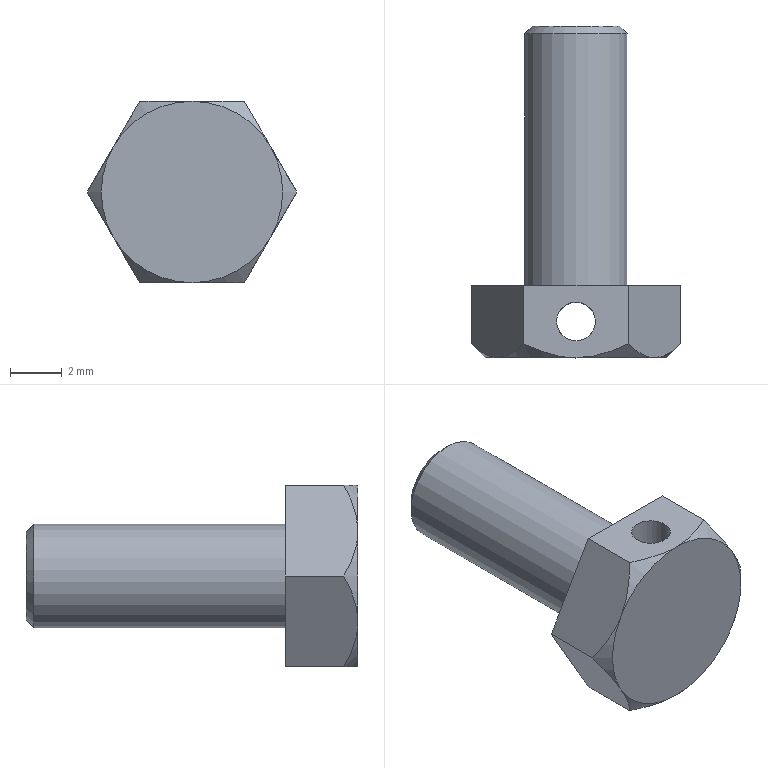Component | NX | BOLT_M4X10 | 1 solid | 18 faces | volume 231 mm3 | plane 9 | cone 7 | cylinder 2 | commonest cylinder face diameters 4 x1 1.5 x1